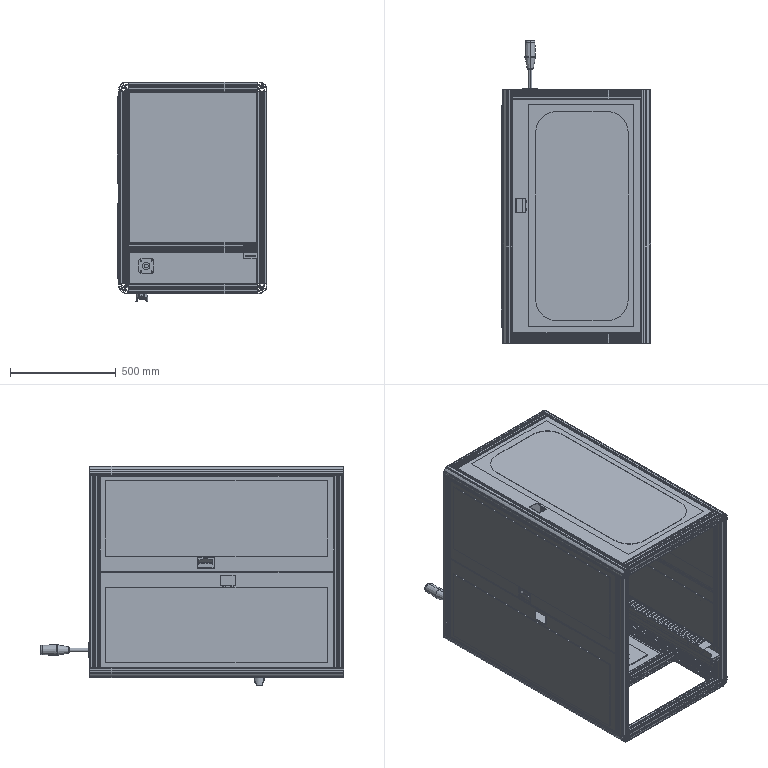Assembly | SolidWorks | mm | 35 component files | 38 solids | 4333 faces | box 707.12 x 1437.15 x 1040 mm | volume 26603364 mm3 | plane 1878 | cylinder 1486 | torus 815 | spline 140 | sphere 8 | cone 6 | commonest cylinder face diameters 2 x626 9.991 x147 3 x124 1 x120 6 x60 1.473 x54 4.473 x52 12.5 x50
Bill of materials:
CAF8-4545-100FF-3 | 6 |  | Long straight square-section extruded bar with a slotted profile: one longitudinal slot centred on each of the four faces, a central round bore with four small lobes, and hollow pockets in the four corners.
CAF8-4545-100GG | 4 |  | Straight square-section slotted extruded bar. Its cross-section matches unnamed part (four side slots, central lobed bore, hollow corners), and it is shown standing vertically.
NFSR8-4545-100AA-2 | 4 |  | Long straight extruded bar with a quarter-round profile. Two adjacent flat faces each carry one longitudinal slot, and the opposite side is a convex arc. Inside are a central bore with one small lobe and several internal cavities.
50MMRodThree-ColorLight | 1 |  | Handle-like part: a square flat base plate with rounded corners and four corner holes, a straight cylindrical shank rising from its centre, and a larger tapered grip with a rounded free end.
BrownAcrylicPlate-2 | 4 |  | Thin flat rectangular plate with no visible holes or cutouts.
BrownAcrylicPlate-4 | 1 |  | Thin flat rectangular sheet, about twice as long as it is wide, with no visible features.
BrownAcrylicPlate-5 | 1 |  | Thin flat rectangular sheet, close to square but slightly longer in one direction, with no visible holes or cutouts.
DoorHandleUWAUNJ80-2 | 1 |  | Small cap- or cover-like part: a thin flange plate with a gently curved top edge and rounded corners, a hollow-looking box body projecting from one face with a rounded upper edge, and two small hook or clip tabs on top.
EmergencyStopButton-0 | 1 |  | Plug-like part: a square block head on a cylindrical stem with two raised ring bands separated by narrower necks, ending in a round flange disc with a slightly domed underside.
EmergencyStopProtectiveCover | 1 |  | Compact block with a rounded-rectangular, partly circular outline. It has a vertical through-bore with two small keyway notches, a large arched saddle cutout through the lower part, and a short open slot on one side.
LEDLightingStrip | 2 |  | Very long, slender rectangular-section strip or bar with a row of small regularly spaced features along its length. One end has small protruding prongs, and the end view shows a rectangle with a rounded lobe on one side.
ElectricalControlMountingPlate | 1 |  | Thin rectangular frame plate with a large central rectangular opening with rounded corners and one small round hole near a corner.
TopPlate | 1 |  | Thin flat rectangular plate. Near one lower corner it has one round through-hole with four small holes around it in a square pattern. Both long side edges have small shallow notches.
UpperDoor1 | 4 |  | Thin flat rectangular frame plate with a large rounded-corner rectangular opening. A small rectangular cutout sits in the wider bottom border strip.
UpperRearDoor | 1 |  | Thin flat rectangular frame plate with a large rounded-corner rectangular (stadium-like) opening. A small rectangular cutout sits in one long side border.
WireDuct1 | 1 |  | Long, narrow bent sheet channel with a U-shaped cross-section: a base web with two upright side walls. At one end the base continues as a flat tab with two small parallel slots. At the other end a tab is bent downward and has an obround slot. Small holes are spaced along the side walls.
WireDuct2 | 1 |  | Long, narrow bent sheet strip with a shallow inverted-U (C) cross-section. The top web has a dense, evenly spaced row of transverse slots with rounded ends. The narrow downturned side flanges each have a few small holes.
Mates:
1. coincident | WireDuct1-1 face at (583, 920, -2103) dir (0, 0, 1) | WireDuct2-1 face at (581, 970, -2103) dir (0, 0, -1)
2. coincident | WireDuct1-1 face at (581, 920, -2103) dir (-1, 0, 0) | WireDuct2-1 face at (581, 970, -2121) dir (1, 0, 0)
3. distance | WireDuct2-1 face at (613, 970, -2111) dir (0, -1, 0) | WireDuct1-1 face at (613, 920, -2120) dir (0, -1, 0)
4. coincident | assembly face at (35, 1220, -1357.5) dir (1, 0, 0) | LEDLightingStrip-1 face at (35, 985, -1357.5) dir (-1, 0, 0)
5. coincident | assembly face at (29, 1220, -1357.5) dir (0, 0, 1) | LEDLightingStrip-1 face at (35, 985, -1357.5) dir (0, 0, 1)
6. distance | 50MMRodThree-ColorLight-1 face at (85, 2124.15, -2235) dir (-1, 0, 0) | assembly face at (35, 2116.15, -1780) dir (1, 0, 0)
7. distance | 50MMRodThree-ColorLight-1 face at (85, 2124.15, -2235) dir (0, 0, -1) | assembly face at (385, 2116.15, -2285) dir (0, 0, 1)
8. parallel | 40-40AluminumProfileFrame-1/CAF8-4545-100FF-3-1 face at (385, 1230, -2312.5) dir (0, -1, 0) | EmergencyStopProtectiveCover-1 face at (98.737, 1342.737, -2370) dir (0, 1, 0)
9. distance | LEDLightingStrip-2 face at (656.5, 985, -2282.5) dir (0, -1, 0) | assembly face at (648, 965, -1780) dir (0, 1, 0)
10. coincident | assembly face at (662.5, 920, -1780) dir (0, -1, 0) | WireDuct1-1 face at (613, 920, -2120) dir (0, -1, 0)
11. coincident | assembly face at (645, 947.5, -1780) dir (-1, 0, 0) | WireDuct1-1 face at (645, 920, -2103) dir (1, 0, 0)
12. distance | LEDLightingStrip-1 face at (37.5, 985, -1363.5) dir (0, -1, 0) | assembly face at (385, 965, -1372) dir (0, 1, 0)
13. coincident | 40-40AluminumProfileFrame-1/NFSR8-4545-100AA-2-1 face at (648, 1220, -2285) dir (0, 0, 1) | LEDLightingStrip-2 face at (650.5, 985, -2285) dir (0, 0, -1)
14. coincident | 40-40AluminumProfileFrame-1/NFSR8-4545-100AA-2-1 face at (662.5, 1220, -2285) dir (1, 0, 0) | LEDLightingStrip-2 face at (662.5, 985, -2285) dir (1, 0, 0)
15. concentric | UpperDoorFrame-1/ElectricalControlMountingPlate-1 face at (98.737, 1318.737, -2325) dir (0, 0, -1) r 11 | EmergencyStopButton-0-1 face at (98.737, 1318.737, -2345.5) dir (0, 0, 1) r 14.5
16. coincident | UpperDoorFrame-1/ElectricalControlMountingPlate-1 face at (435, 1924.15, -2330) dir (0, 0, -1) | EmergencyStopProtectiveCover-1 face at (98.737, 1318.737, -2330) dir (0, 0, 1)
17. coincident | UpperDoorFrame-1/TopPlate-1 face at (245, 2119.15, -1785) dir (0, 1, 0) | 50MMRodThree-ColorLight-1 face at (120, 2119.15, -2200) dir (0, -1, 0)
18. coincident | UpperDoorFrame-1/UpperRearDoor-1 face at (444.5, 1767.65, -1331.5) dir (0, 0, -1) | BrownAcrylicPlate-5/BrownAcrylicPlate-4-1 face at (360.5, 1525.65, -1331.5) dir (0, 0, 1)
19. distance | UpperDoorFrame-1/UpperRearDoor-1 face at (483.5, 2015.65, -1321.5) dir (0, -1, 0) | BrownAcrylicPlate-5/BrownAcrylicPlate-4-1 face at (110.5, 2050.65, -1331.5) dir (0, 1, 0)
20. distance | BrownAcrylicPlate-5/BrownAcrylicPlate-4-1 face at (110.5, 2050.65, -1331.5) dir (-1, 0, 0) | UpperDoorFrame-1/UpperRearDoor-1 face at (145.5, 1915.65, -1321.5) dir (1, 0, 0)
21. coincident | UpperDoorFrame-1/ElectricalControlMountingPlate-1 face at (435, 1924.15, -2328.5) dir (0, 0, 1) | BrownAcrylicPlate-5/BrownAcrylicPlate-5-1 face at (335.689, 1675.552, -2328.5) dir (0, 0, -1)
22. concentric | EmergencyStopButton-0-1 face at (98.737, 1318.737, -2345.5) dir (0, 0, 1) r 14.5 | EmergencyStopProtectiveCover-1 face at (98.737, 1318.737, -2331.5) dir (0, 0, 1) r 11
23. distance | UpperDoorFrame-1/ElectricalControlMountingPlate-1 face at (435, 1924.15, -2330) dir (0, 0, -1) | EmergencyStopButton-0-1 face at (113.817, 1303.642, -2331.5) dir (0, 0, 1)
24. coincident | CAF8-4545-100FF-3-2 face at (385, 920, -2312.5) dir (0, -1, 0) | NFSR8-4545-100AA-2-2 face at (-9, 920, -2286) dir (0, -1, 0)
25. coincident | NFSR8-4545-100AA-2-1 face at (646, 920, -2329) dir (0, -1, 0) | CAF8-4545-100FF-3-2 face at (385, 920, -2312.5) dir (0, -1, 0)
26. coincident | CAF8-4545-100FF-3-2 face at (35, 923, -2288) dir (-1, 0, 0) | NFSR8-4545-100AA-2-2 face at (35, 1220, -2288) dir (1, 0, 0)
27. coincident | CAF8-4545-100FF-3-3 face at (35, 923, -1333) dir (-1, 0, 0) | NFSR8-4545-100AA-2-3 face at (35, 1220, -1331) dir (1, 0, 0)
28. coincident | CAF8-4545-100FF-3-3 face at (645, 923, -1333) dir (1, 0, 0) | NFSR8-4545-100AA-2-4 face at (645, 1220, -1347.5) dir (-1, 0, 0)
29. coincident | CAF8-4545-100FF-3-2 face at (385, 965, -2327) dir (0, 1, 0) | CAF8-4545-100GG-6 face at (648, 965, -1780) dir (0, 1, 0)
30. coincident | NFSR8-4545-100AA-2-1 face at (690, 1220, -2286) dir (1, 0, 0) | CAF8-4545-100GG-6 face at (690, 962, -1780) dir (1, 0, 0)
31. coincident | NFSR8-4545-100AA-2-4 face at (689, 1220, -1375) dir (0, 0, -1) | CAF8-4545-100GG-6 face at (648, 962, -1375) dir (0, 0, 1)
32. coincident | CAF8-4545-100FF-3-3 face at (385, 965, -1372) dir (0, 1, 0) | CAF8-4545-100GG-7 face at (-7, 965, -1780) dir (0, 1, 0)
33. coincident | NFSR8-4545-100AA-2-3 face at (7.5, 1220, -1375) dir (0, 0, -1) | CAF8-4545-100GG-7 face at (-7, 962, -1375) dir (0, 0, 1)
34. coincident | NFSR8-4545-100AA-2-3 face at (-10, 1220, -1374) dir (-1, 0, 0) | CAF8-4545-100GG-7 face at (-10, 923, -1780) dir (-1, 0, 0)
35. coincident | CAF8-4545-100FF-3-4 face at (385, 2119.15, -1372) dir (0, 1, 0) | CAF8-4545-100GG-4 face at (17.5, 2119.15, -1780) dir (0, 1, 0)
36. coincident | NFSR8-4545-100AA-2-3 face at (-10, 1220, -1374) dir (-1, 0, 0) | CAF8-4545-100GG-4 face at (-10, 2101.65, -1780) dir (-1, 0, 0)
37. coincident | NFSR8-4545-100AA-2-3 face at (7.5, 1220, -1375) dir (0, 0, -1) | CAF8-4545-100GG-4 face at (-7, 2116.15, -1375) dir (0, 0, 1)
38. coincident | CAF8-4545-100GG-5 face at (645, 2101.65, -1780) dir (-1, 0, 0) | CAF8-4545-100FF-3-6 face at (645, 2075.65, -2093) dir (1, 0, 0)
39. distance | CAF8-4545-100FF-3-5 face at (385, 2116.15, -2285) dir (0, 0, 1) | CAF8-4545-100FF-3-6 face at (385, 2100.15, -2135) dir (0, 0, -1)
40. distance | CAF8-4545-100GG-5 face at (648, 2119.15, -1780) dir (0, 1, 0) | CAF8-4545-100FF-3-6 face at (385, 2117.65, -2132) dir (0, 1, 0)
41. coincident | UpperDoor1-1 face at (-10, 1767.65, -1580.5) dir (-1, 0, 0) | UpperDoor1-4 face at (-10, 1271.5, -2079.5) dir (-1, 0, 0)
42. coincident | UpperDoor1-1 face at (-8.5, 2072.65, -1580.5) dir (0, 1, 0) | UpperDoor1-4 face at (-8.5, 2072.65, -2079.5) dir (0, 1, 0)
43. coincident | TopPlate-1 face at (245, 2117.65, -2283.5) dir (0, 0, -1) | UpperDoor1-4 face at (-8.5, 1271.5, -2283.5) dir (0, 0, -1)
44. distance | UpperDoor1-2 face at (690, 1271.5, -1580.5) dir (1, 0, 0) | TopPlate-1 face at (643.5, 2117.65, -1785) dir (1, 0, 0)
45. coincident | TopPlate-1 face at (245, 2117.65, -1376.5) dir (0, 0, 1) | UpperDoor1-2 face at (688.5, 1271.5, -1376.5) dir (0, 0, 1)
46. coincident | UpperDoor1-2 face at (690, 1271.5, -1580.5) dir (1, 0, 0) | UpperDoor1-3 face at (690, 1767.65, -2079.5) dir (1, 0, 0)
47. coincident | TopPlate-1 face at (245, 2117.65, -2283.5) dir (0, 0, -1) | UpperDoor1-3 face at (688.5, 1767.65, -2283.5) dir (0, 0, -1)
48. coincident | UpperDoor1-2 face at (688.5, 2072.65, -1580.5) dir (0, 1, 0) | UpperDoor1-3 face at (688.5, 2072.65, -2079.5) dir (0, 1, 0)
49. coincident | ElectricalControlMountingPlate-1 face at (435, 2072.65, -2328.5) dir (0, 1, 0) | UpperDoor1-3 face at (688.5, 2072.65, -2079.5) dir (0, 1, 0)